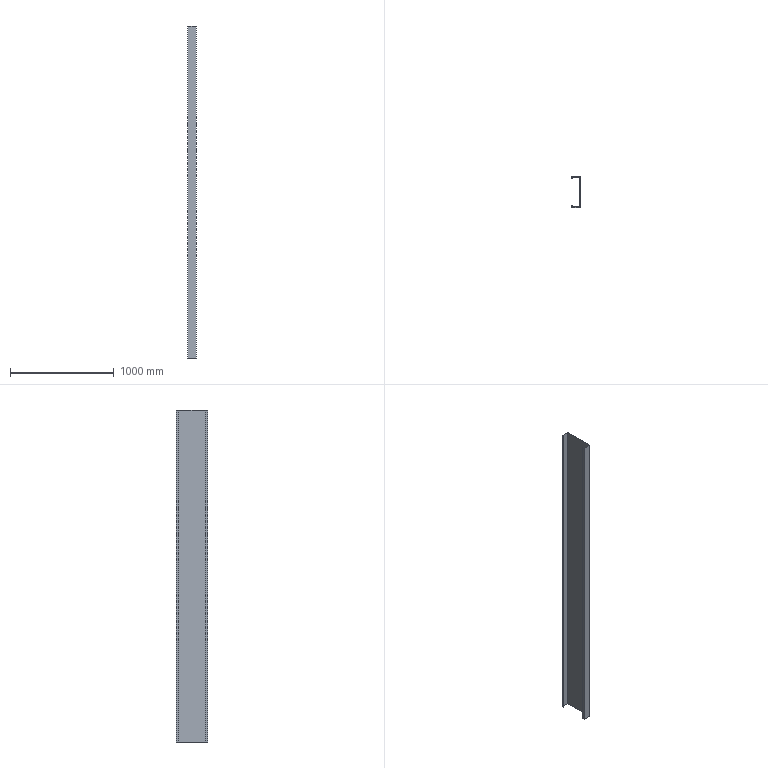Component | NX | CBLIANJIE_13 | 1 solid | 14 faces | volume 4677480 mm3 | plane 14